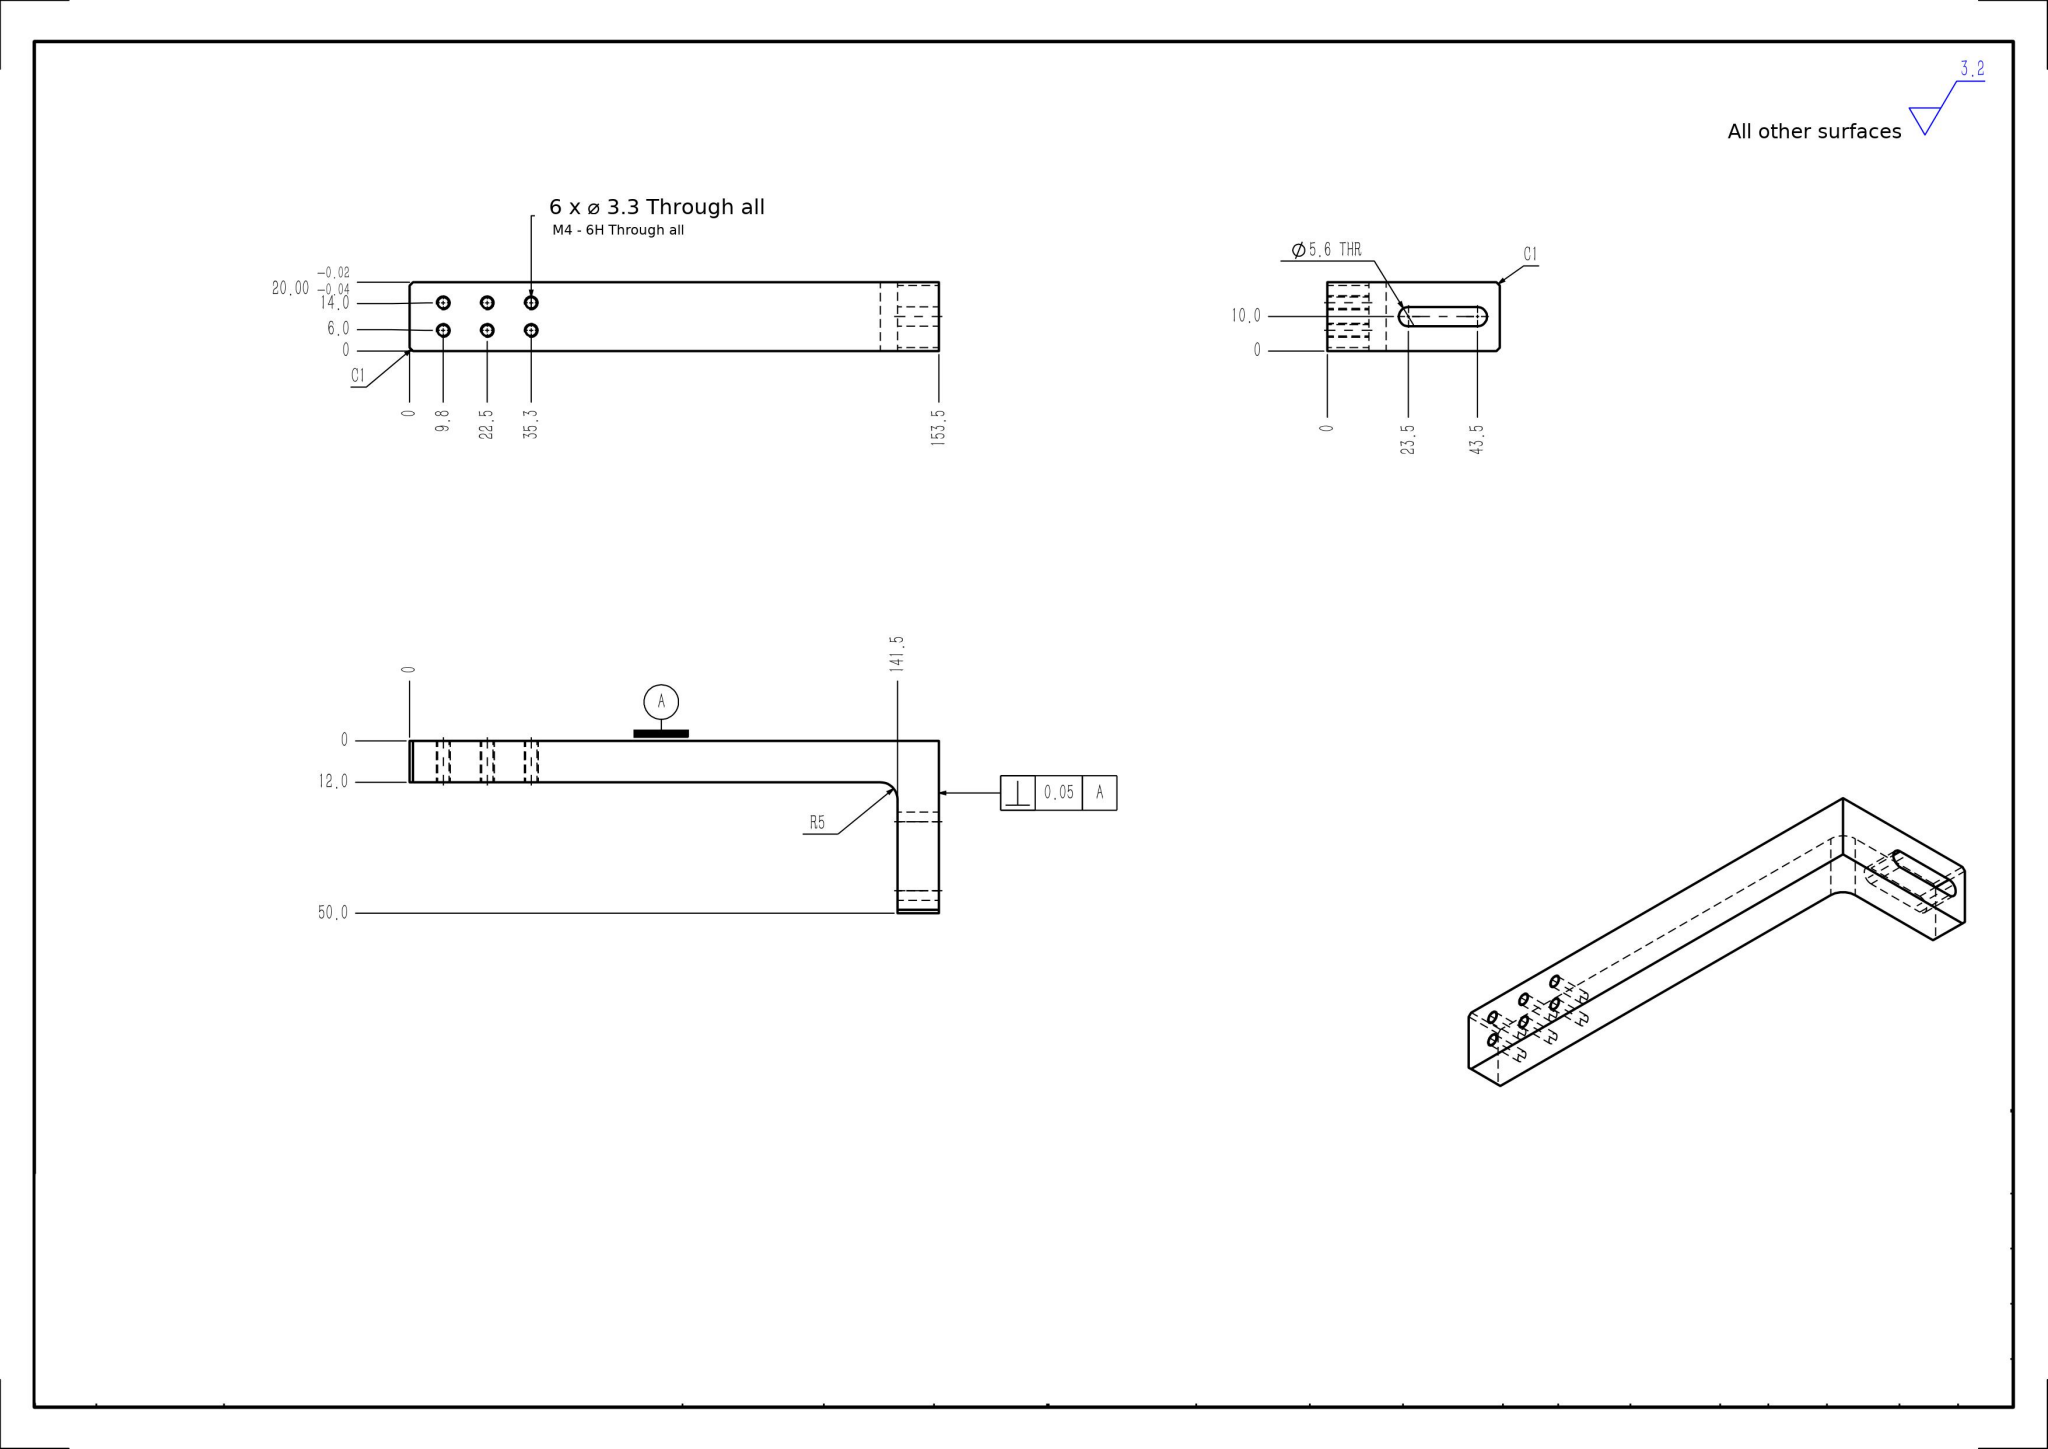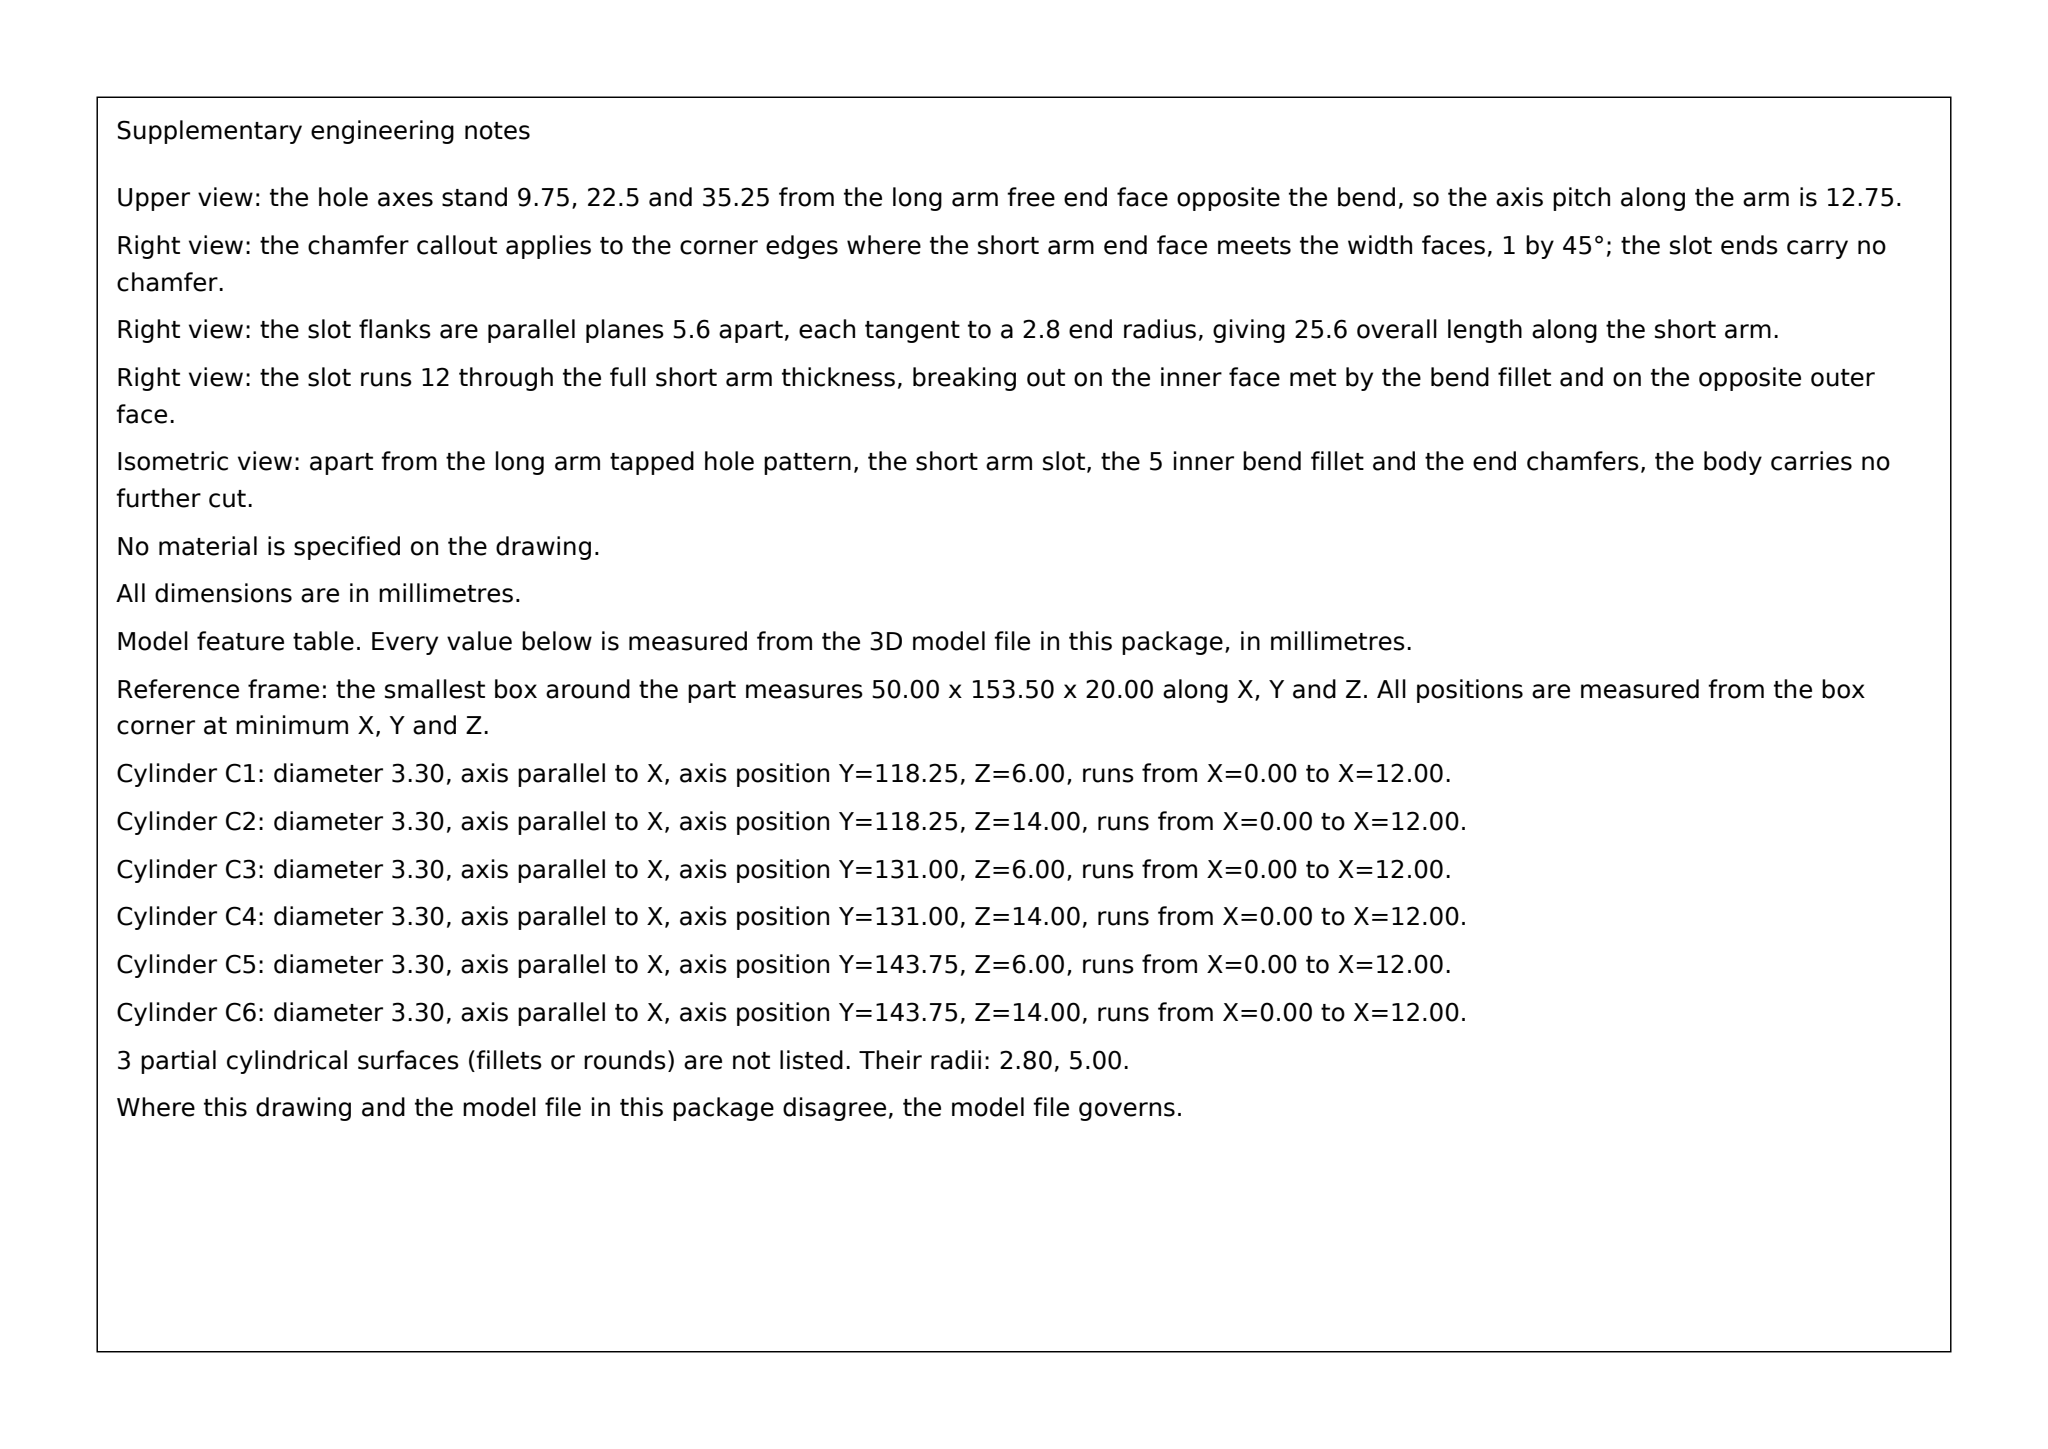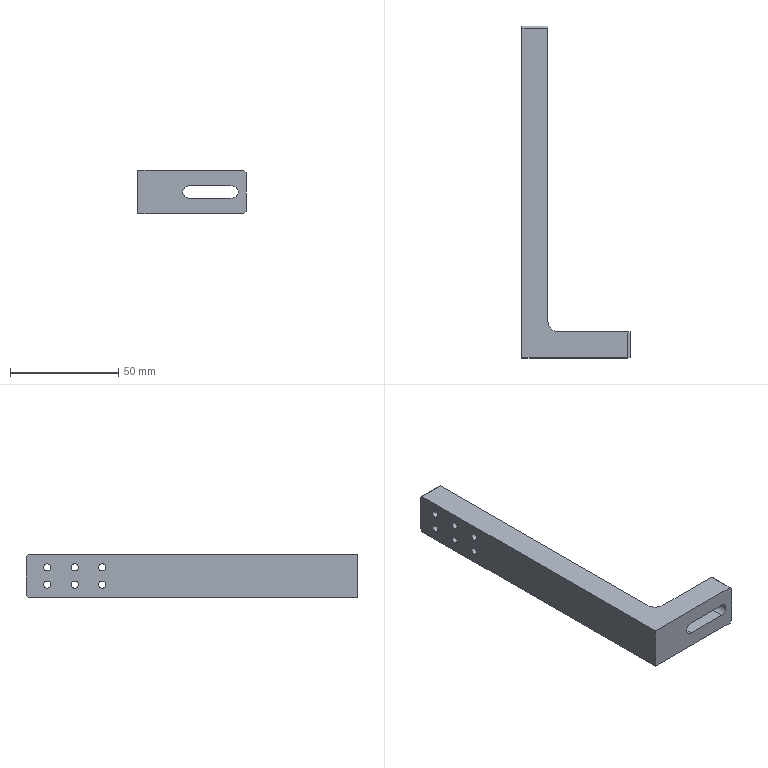Part | SolidWorks | mm | 1 solid | 30 faces | box 50 x 153.5 x 20 mm | volume 43788 mm3 | cylinder 16 | plane 14 | commonest cylinder face diameters 3.3 x12 5.6 x3 10 x1
Drawing notes:
Ø5.6 THRU (12 THK WALL); SLOT CTRS 23.5 & 43.5 | from the solid: cyl dia 5.6, axis y, length 12 = wall thk (y 0 to 12), centers at x=23.5 and 43.5, z=10.0
build123d program:
from build123d import *

# Parameters (mm, degrees)
BOSS_EXTRUDE1_DEPTH = 10
FILLET1_R           = 5
CUT_EXTRUDE1_DEPTH  = 145.039
CHAMFER1_SIZE       = 1
M4_TAPPED_HOLE1_D   = 3.3


with BuildPart() as part:
    # Sketch1 → Boss-Extrude1 (new, symmetric)
    with BuildSketch(Plane.XY):
        Polygon((-13, 76.75), (-13, -64.75), (25, -64.75), (25, -76.75), (-25, -76.75), (-25, 76.75), align=None)
    extrude(amount=BOSS_EXTRUDE1_DEPTH, both=True)

    # Fillet1
    fillet1_edges = [part.edges().sort_by_distance(p)[0] for p in [
        (-13, -64.75, 0),
    ]]
    fillet(fillet1_edges, radius=FILLET1_R)

    # Sketch2 → Cut-Extrude1 (cut, through all)
    with BuildSketch(Plane(origin=(0, -64.75, 0), x_dir=(1, 0, 0), z_dir=(0, 1, 0))):
        with BuildLine():
            Line((-1.5, 2.8), (18.5, 2.8))
            ThreePointArc((18.5, 2.8), (21.3, 0), (18.5, -2.8))
            Line((18.5, -2.8), (-1.5, -2.8))
            ThreePointArc((-1.5, -2.8), (-4.3, 0), (-1.5, 2.8))
        make_face()
    extrude(amount=-CUT_EXTRUDE1_DEPTH, mode=Mode.SUBTRACT)

    # Chamfer1
    chamfer1_edges = [part.edges().sort_by_distance(p)[0] for p in [
        (25, -70.75, 10),
        (-19, 76.75, 10),
        (-19, 76.75, -10),
        (25, -70.75, -10),
    ]]
    chamfer(chamfer1_edges, length=CHAMFER1_SIZE)

    # M4 Tapped Hole1 (through all)
    with Locations(Plane.ZY.offset(25)):
        with Locations((-4, 67), (-4, 41.5), (-4, 54.25), (4, 41.5), (4, 54.25), (4, 67)):
            Hole(M4_TAPPED_HOLE1_D / 2)


solid = part.part